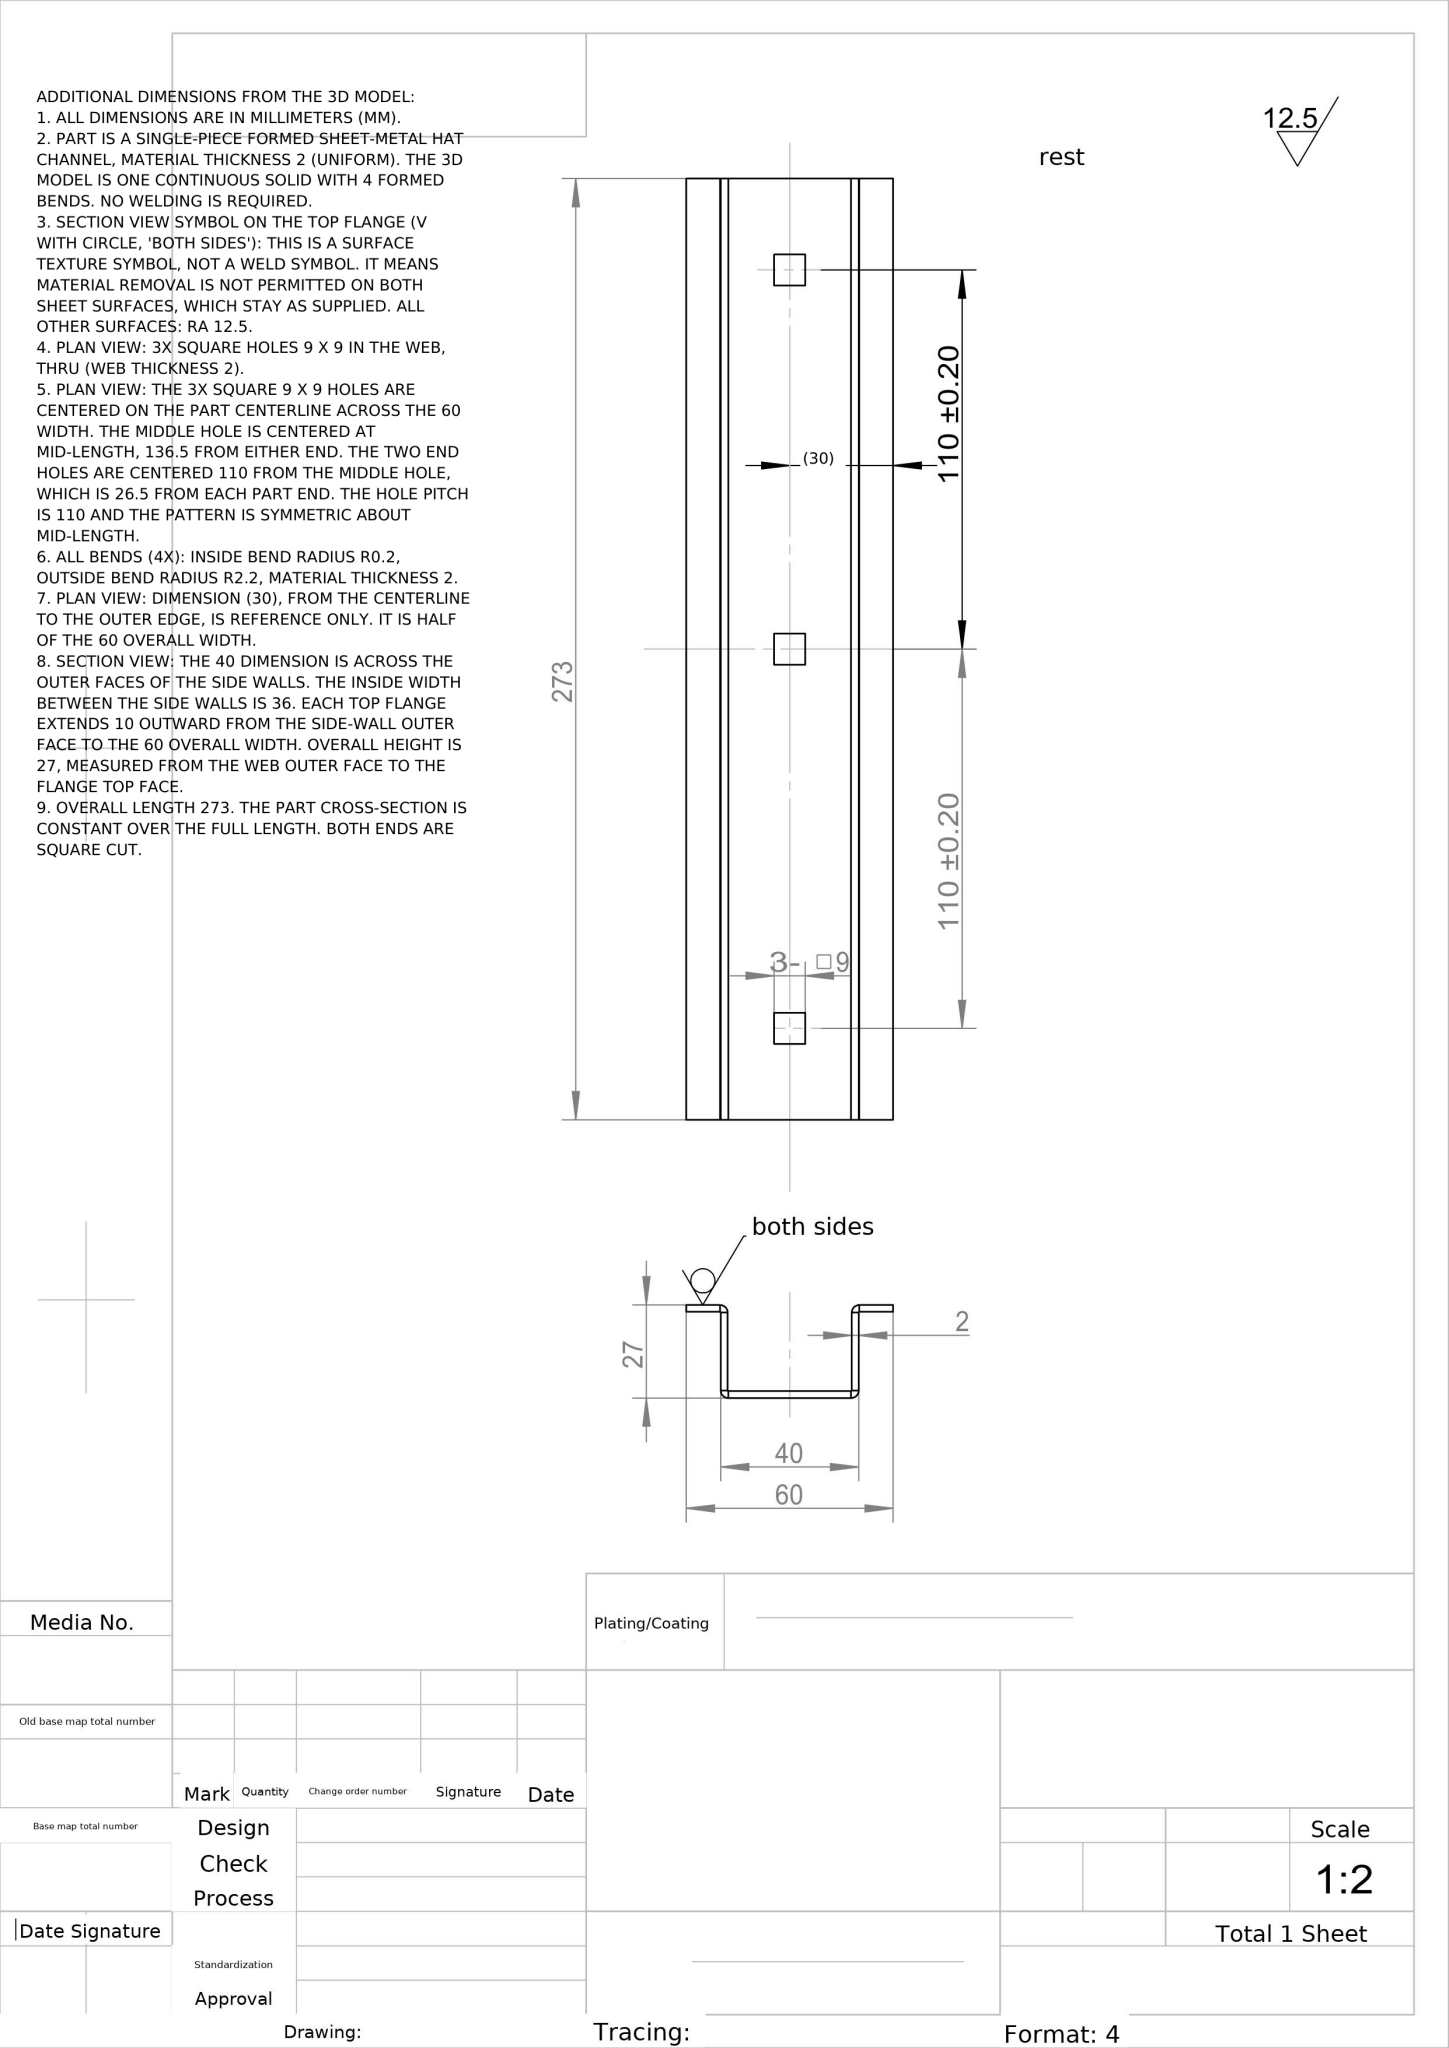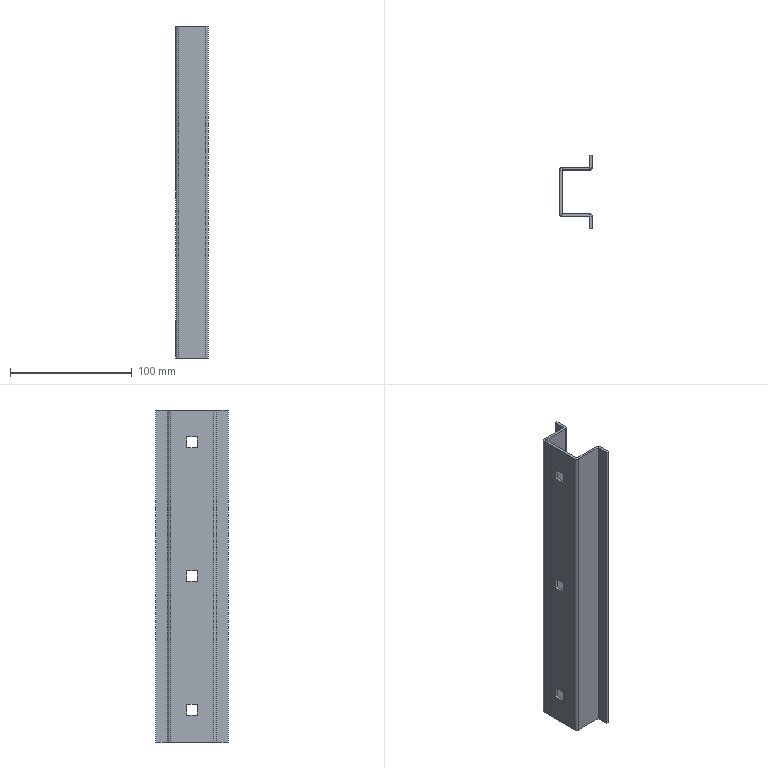Part | NX | mm | 1 solid | 50 faces | box 27 x 60 x 273 mm | volume 58449 mm3 | plane 42 | cylinder 8 | commonest cylinder face diameters 0.4 x4 4.4 x4